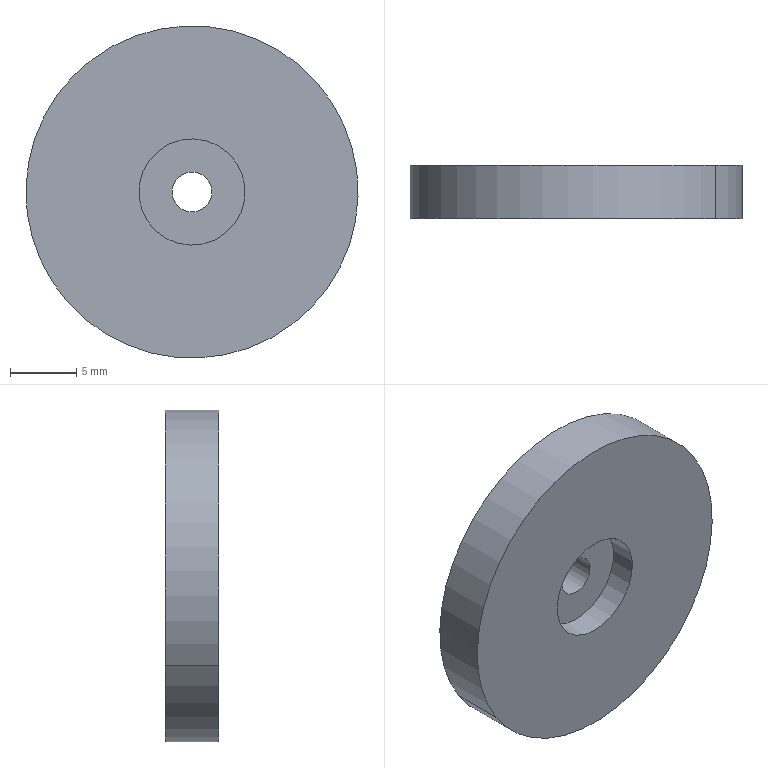Component | SolidWorks | EndCap4mm-3 | 1 solid | 9 faces | box 25 x 4 x 25 mm | volume 1849 mm3 | cylinder 6 | plane 3 | commonest cylinder face diameters 8 x2 25 x2 3 x2 | material 5454-O
build123d program:
from build123d import *

# Parameters (mm, degrees)
SKETCH1_R           = 12.5
SKETCH1_R_2         = 1.5
BOSS_EXTRUDE1_DEPTH = 4
SKETCH2_R           = 4
CUT_EXTRUDE1_DEPTH  = 2


with BuildPart() as part:
    # Sketch1 → Boss-Extrude1 (new body)
    with BuildSketch(Plane.XY):
        Circle(SKETCH1_R)
        Circle(SKETCH1_R_2, mode=Mode.SUBTRACT)
    extrude(amount=BOSS_EXTRUDE1_DEPTH)

    # Sketch2 → Cut-Extrude1 (cut)
    with BuildSketch(Plane.XY.offset(4)):
        Circle(SKETCH2_R)
    extrude(amount=-CUT_EXTRUDE1_DEPTH, mode=Mode.SUBTRACT)


solid = part.part

# Placed as in the assembly
solid = solid.moved(Location((6.846, 48.266, -166.507), (90, 0, 0)))
STEP:
#1=COLOUR_RGB('',0.7922,0.8196,0.9333);
#2=FILL_AREA_STYLE_COLOUR('',#1);
#3=FILL_AREA_STYLE('',(#2));
#4=SURFACE_STYLE_FILL_AREA(#3);
#5=SURFACE_SIDE_STYLE('',(#4));
#6=SURFACE_STYLE_USAGE(.BOTH.,#5);
#7=PRESENTATION_STYLE_ASSIGNMENT((#6));
#8=CARTESIAN_POINT('',(0.137,1.821,-6.641));
#9=VERTEX_POINT('',#8);
#10=CARTESIAN_POINT('',(0.402,1.821,-6.47));
#11=VERTEX_POINT('',#10);
#12=CARTESIAN_POINT('',(0.2695,1.821,-6.555));
#13=DIRECTION('',(-0.,-1.,-0.));
#14=DIRECTION('',(0.8414,0.,0.5405));
#15=AXIS2_PLACEMENT_3D('',#12,#13,#14);
#16=CIRCLE('',#15,0.1575);
#17=EDGE_CURVE('',#9,#11,#16,.T.);
#18=ORIENTED_EDGE('',*,*,#17,.F.);
#19=CARTESIAN_POINT('',(0.137,1.743,-6.641));
#20=VERTEX_POINT('',#19);
#21=CARTESIAN_POINT('',(0.137,1.821,-6.641));
#22=DIRECTION('',(-0.,-1.,-0.));
#23=VECTOR('',#22,39.37);
#24=LINE('',#21,#23);
#25=EDGE_CURVE('',#9,#20,#24,.T.);
#26=ORIENTED_EDGE('',*,*,#25,.T.);
#27=CARTESIAN_POINT('',(0.402,1.743,-6.47));
#28=VERTEX_POINT('',#27);
#29=CARTESIAN_POINT('',(0.2695,1.743,-6.555));
#30=DIRECTION('',(-0.,-1.,-0.));
#31=DIRECTION('',(0.8414,0.,0.5405));
#32=AXIS2_PLACEMENT_3D('',#29,#30,#31);
#33=CIRCLE('',#32,0.1575);
#34=EDGE_CURVE('',#20,#28,#33,.T.);
#35=ORIENTED_EDGE('',*,*,#34,.T.);
#36=CARTESIAN_POINT('',(0.402,1.821,-6.47));
#37=DIRECTION('',(-0.,-1.,-0.));
#38=VECTOR('',#37,39.37);
#39=LINE('',#36,#38);
#40=EDGE_CURVE('',#11,#28,#39,.T.);
#41=ORIENTED_EDGE('',*,*,#40,.F.);
#42=EDGE_LOOP('',(#18,#26,#35,#41));
#43=FACE_OUTER_BOUND('',#42,.T.);
#44=CARTESIAN_POINT('',(0.2695,1.821,-6.555));
#45=DIRECTION('',(-0.,-1.,-0.));
#46=DIRECTION('',(0.8414,0.,0.5405));
#47=AXIS2_PLACEMENT_3D('',#44,#45,#46);
#48=CYLINDRICAL_SURFACE('',#47,0.1575);
#49=ADVANCED_FACE('',(#43),#48,.F.);
#50=CARTESIAN_POINT('',(0.6836,1.743,-6.289));
#51=VERTEX_POINT('',#50);
#52=CARTESIAN_POINT('',(-0.1445,1.743,-6.821));
#53=VERTEX_POINT('',#52);
#54=CARTESIAN_POINT('',(0.2695,1.743,-6.555));
#55=DIRECTION('',(-0.,-1.,-0.));
#56=DIRECTION('',(0.8414,0.,0.5405));
#57=AXIS2_PLACEMENT_3D('',#54,#55,#56);
#58=CIRCLE('',#57,0.4921);
#59=EDGE_CURVE('',#51,#53,#58,.T.);
#60=ORIENTED_EDGE('',*,*,#59,.F.);
#61=CARTESIAN_POINT('',(0.6836,1.9,-6.289));
#62=VERTEX_POINT('',#61);
#63=CARTESIAN_POINT('',(0.6836,1.743,-6.289));
#64=DIRECTION('',(0.,1.,0.));
#65=VECTOR('',#64,39.37);
#66=LINE('',#63,#65);
#67=EDGE_CURVE('',#51,#62,#66,.T.);
#68=ORIENTED_EDGE('',*,*,#67,.T.);
#69=CARTESIAN_POINT('',(-0.1445,1.9,-6.821));
#70=VERTEX_POINT('',#69);
#71=CARTESIAN_POINT('',(0.2695,1.9,-6.555));
#72=DIRECTION('',(-0.,-1.,-0.));
#73=DIRECTION('',(0.8414,0.,0.5405));
#74=AXIS2_PLACEMENT_3D('',#71,#72,#73);
#75=CIRCLE('',#74,0.4921);
#76=EDGE_CURVE('',#62,#70,#75,.T.);
#77=ORIENTED_EDGE('',*,*,#76,.T.);
#78=CARTESIAN_POINT('',(-0.1445,1.743,-6.821));
#79=DIRECTION('',(0.,1.,0.));
#80=VECTOR('',#79,39.37);
#81=LINE('',#78,#80);
#82=EDGE_CURVE('',#53,#70,#81,.T.);
#83=ORIENTED_EDGE('',*,*,#82,.F.);
#84=EDGE_LOOP('',(#60,#68,#77,#83));
#85=FACE_OUTER_BOUND('',#84,.T.);
#86=CARTESIAN_POINT('',(0.2695,1.743,-6.555));
#87=DIRECTION('',(0.,1.,0.));
#88=DIRECTION('',(-0.8414,0.,-0.5405));
#89=AXIS2_PLACEMENT_3D('',#86,#87,#88);
#90=CYLINDRICAL_SURFACE('',#89,0.4921);
#91=ADVANCED_FACE('',(#85),#90,.T.);
#92=CARTESIAN_POINT('',(0.2198,1.821,-6.587));
#93=VERTEX_POINT('',#92);
#94=CARTESIAN_POINT('',(0.3192,1.821,-6.523));
#95=VERTEX_POINT('',#94);
#96=CARTESIAN_POINT('',(0.2695,1.821,-6.555));
#97=DIRECTION('',(-0.,-1.,-0.));
#98=DIRECTION('',(0.8414,0.,0.5405));
#99=AXIS2_PLACEMENT_3D('',#96,#97,#98);
#100=CIRCLE('',#99,0.05906);
#101=EDGE_CURVE('',#93,#95,#100,.T.);
#102=ORIENTED_EDGE('',*,*,#101,.T.);
#103=CARTESIAN_POINT('',(0.3192,1.9,-6.523));
#104=VERTEX_POINT('',#103);
#105=CARTESIAN_POINT('',(0.3192,1.743,-6.523));
#106=DIRECTION('',(0.,1.,0.));
#107=VECTOR('',#106,39.37);
#108=LINE('',#105,#107);
#109=EDGE_CURVE('',#95,#104,#108,.T.);
#110=ORIENTED_EDGE('',*,*,#109,.T.);
#111=CARTESIAN_POINT('',(0.2198,1.9,-6.587));
#112=VERTEX_POINT('',#111);
#113=CARTESIAN_POINT('',(0.2695,1.9,-6.555));
#114=DIRECTION('',(-0.,-1.,-0.));
#115=DIRECTION('',(0.8414,0.,0.5405));
#116=AXIS2_PLACEMENT_3D('',#113,#114,#115);
#117=CIRCLE('',#116,0.05906);
#118=EDGE_CURVE('',#112,#104,#117,.T.);
#119=ORIENTED_EDGE('',*,*,#118,.F.);
#120=CARTESIAN_POINT('',(0.2198,1.743,-6.587));
#121=DIRECTION('',(0.,1.,0.));
#122=VECTOR('',#121,39.37);
#123=LINE('',#120,#122);
#124=EDGE_CURVE('',#93,#112,#123,.T.);
#125=ORIENTED_EDGE('',*,*,#124,.F.);
#126=EDGE_LOOP('',(#102,#110,#119,#125));
#127=FACE_OUTER_BOUND('',#126,.T.);
#128=CARTESIAN_POINT('',(0.2695,1.743,-6.555));
#129=DIRECTION('',(0.,1.,0.));
#130=DIRECTION('',(-0.8414,0.,-0.5405));
#131=AXIS2_PLACEMENT_3D('',#128,#129,#130);
#132=CYLINDRICAL_SURFACE('',#131,0.05906);
#133=ADVANCED_FACE('',(#127),#132,.F.);
#134=ORIENTED_EDGE('',*,*,#109,.F.);
#135=CARTESIAN_POINT('',(0.2695,1.821,-6.555));
#136=DIRECTION('',(-0.,-1.,-0.));
#137=DIRECTION('',(0.8414,0.,0.5405));
#138=AXIS2_PLACEMENT_3D('',#135,#136,#137);
#139=CIRCLE('',#138,0.05906);
#140=EDGE_CURVE('',#95,#93,#139,.T.);
#141=ORIENTED_EDGE('',*,*,#140,.T.);
#142=ORIENTED_EDGE('',*,*,#124,.T.);
#143=CARTESIAN_POINT('',(0.2695,1.9,-6.555));
#144=DIRECTION('',(-0.,-1.,-0.));
#145=DIRECTION('',(0.8414,0.,0.5405));
#146=AXIS2_PLACEMENT_3D('',#143,#144,#145);
#147=CIRCLE('',#146,0.05906);
#148=EDGE_CURVE('',#104,#112,#147,.T.);
#149=ORIENTED_EDGE('',*,*,#148,.F.);
#150=EDGE_LOOP('',(#134,#141,#142,#149));
#151=FACE_OUTER_BOUND('',#150,.T.);
#152=CARTESIAN_POINT('',(0.2695,1.743,-6.555));
#153=DIRECTION('',(0.,1.,0.));
#154=DIRECTION('',(-0.8414,0.,-0.5405));
#155=AXIS2_PLACEMENT_3D('',#152,#153,#154);
#156=CYLINDRICAL_SURFACE('',#155,0.05906);
#157=ADVANCED_FACE('',(#151),#156,.F.);
#158=CARTESIAN_POINT('',(0.2695,1.743,-6.555));
#159=DIRECTION('',(-0.,-1.,-0.));
#160=DIRECTION('',(0.8414,0.,0.5405));
#161=AXIS2_PLACEMENT_3D('',#158,#159,#160);
#162=CIRCLE('',#161,0.1575);
#163=EDGE_CURVE('',#28,#20,#162,.T.);
#164=ORIENTED_EDGE('',*,*,#163,.F.);
#165=ORIENTED_EDGE('',*,*,#34,.F.);
#166=EDGE_LOOP('',(#164,#165));
#167=FACE_BOUND('',#166,.T.);
#168=CARTESIAN_POINT('',(0.2695,1.743,-6.555));
#169=DIRECTION('',(-0.,-1.,-0.));
#170=DIRECTION('',(0.8414,0.,0.5405));
#171=AXIS2_PLACEMENT_3D('',#168,#169,#170);
#172=CIRCLE('',#171,0.4921);
#173=EDGE_CURVE('',#53,#51,#172,.T.);
#174=ORIENTED_EDGE('',*,*,#173,.T.);
#175=ORIENTED_EDGE('',*,*,#59,.T.);
#176=EDGE_LOOP('',(#174,#175));
#177=FACE_OUTER_BOUND('',#176,.T.);
#178=CARTESIAN_POINT('',(0.2695,1.743,-6.555));
#179=DIRECTION('',(-0.,-1.,-0.));
#180=DIRECTION('',(0.8414,-0.,0.5405));
#181=AXIS2_PLACEMENT_3D('',#178,#179,#180);
#182=PLANE('',#181);
#183=ADVANCED_FACE('',(#167,#177),#182,.T.);
#184=CARTESIAN_POINT('',(0.2695,1.9,-6.555));
#185=DIRECTION('',(-0.,-1.,-0.));
#186=DIRECTION('',(0.8414,0.,0.5405));
#187=AXIS2_PLACEMENT_3D('',#184,#185,#186);
#188=CIRCLE('',#187,0.4921);
#189=EDGE_CURVE('',#70,#62,#188,.T.);
#190=ORIENTED_EDGE('',*,*,#189,.F.);
#191=ORIENTED_EDGE('',*,*,#76,.F.);
#192=EDGE_LOOP('',(#190,#191));
#193=FACE_OUTER_BOUND('',#192,.T.);
#194=ORIENTED_EDGE('',*,*,#118,.T.);
#195=ORIENTED_EDGE('',*,*,#148,.T.);
#196=EDGE_LOOP('',(#194,#195));
#197=FACE_BOUND('',#196,.T.);
#198=CARTESIAN_POINT('',(0.2695,1.9,-6.555));
#199=DIRECTION('',(-0.,-1.,-0.));
#200=DIRECTION('',(0.8414,-0.,0.5405));
#201=AXIS2_PLACEMENT_3D('',#198,#199,#200);
#202=PLANE('',#201);
#203=ADVANCED_FACE('',(#193,#197),#202,.F.);
#204=ORIENTED_EDGE('',*,*,#67,.F.);
#205=ORIENTED_EDGE('',*,*,#173,.F.);
#206=ORIENTED_EDGE('',*,*,#82,.T.);
#207=ORIENTED_EDGE('',*,*,#189,.T.);
#208=EDGE_LOOP('',(#204,#205,#206,#207));
#209=FACE_OUTER_BOUND('',#208,.T.);
#210=CARTESIAN_POINT('',(0.2695,1.743,-6.555));
#211=DIRECTION('',(0.,1.,0.));
#212=DIRECTION('',(-0.8414,0.,-0.5405));
#213=AXIS2_PLACEMENT_3D('',#210,#211,#212);
#214=CYLINDRICAL_SURFACE('',#213,0.4921);
#215=ADVANCED_FACE('',(#209),#214,.T.);
#216=ORIENTED_EDGE('',*,*,#25,.F.);
#217=CARTESIAN_POINT('',(0.2695,1.821,-6.555));
#218=DIRECTION('',(-0.,-1.,-0.));
#219=DIRECTION('',(0.8414,0.,0.5405));
#220=AXIS2_PLACEMENT_3D('',#217,#218,#219);
#221=CIRCLE('',#220,0.1575);
#222=EDGE_CURVE('',#11,#9,#221,.T.);
#223=ORIENTED_EDGE('',*,*,#222,.F.);
#224=ORIENTED_EDGE('',*,*,#40,.T.);
#225=ORIENTED_EDGE('',*,*,#163,.T.);
#226=EDGE_LOOP('',(#216,#223,#224,#225));
#227=FACE_OUTER_BOUND('',#226,.T.);
#228=CARTESIAN_POINT('',(0.2695,1.821,-6.555));
#229=DIRECTION('',(-0.,-1.,-0.));
#230=DIRECTION('',(0.8414,0.,0.5405));
#231=AXIS2_PLACEMENT_3D('',#228,#229,#230);
#232=CYLINDRICAL_SURFACE('',#231,0.1575);
#233=ADVANCED_FACE('',(#227),#232,.F.);
#234=ORIENTED_EDGE('',*,*,#101,.F.);
#235=ORIENTED_EDGE('',*,*,#140,.F.);
#236=EDGE_LOOP('',(#234,#235));
#237=FACE_BOUND('',#236,.T.);
#238=ORIENTED_EDGE('',*,*,#222,.T.);
#239=ORIENTED_EDGE('',*,*,#17,.T.);
#240=EDGE_LOOP('',(#238,#239));
#241=FACE_OUTER_BOUND('',#240,.T.);
#242=CARTESIAN_POINT('',(0.2695,1.821,-6.555));
#243=DIRECTION('',(-0.,-1.,-0.));
#244=DIRECTION('',(0.8414,-0.,0.5405));
#245=AXIS2_PLACEMENT_3D('',#242,#243,#244);
#246=PLANE('',#245);
#247=ADVANCED_FACE('',(#237,#241),#246,.T.);
#248=CLOSED_SHELL('',(#49,#91,#133,#157,#183,#203,#215,#233,#247));
#249=MANIFOLD_SOLID_BREP('',#248);
#250=STYLED_ITEM('',(#7),#249);
#251=(LENGTH_UNIT()NAMED_UNIT(*)SI_UNIT($,.METRE.));
#252=LENGTH_MEASURE_WITH_UNIT(LENGTH_MEASURE(0.0254),#251);
#253=DIMENSIONAL_EXPONENTS(1.,0.,0.,0.,0.,0.,0.);
#254=(CONVERSION_BASED_UNIT('',#252)LENGTH_UNIT()NAMED_UNIT(#253));
#255=UNCERTAINTY_MEASURE_WITH_UNIT(LENGTH_MEASURE(0.00001),#254,'','');
#256=(NAMED_UNIT(*)PLANE_ANGLE_UNIT()SI_UNIT($,.RADIAN.));
#257=(NAMED_UNIT(*)SI_UNIT($,.STERADIAN.)SOLID_ANGLE_UNIT());
#258=(GEOMETRIC_REPRESENTATION_CONTEXT(3)GLOBAL_UNCERTAINTY_ASSIGNED_CONTEXT((#255))GLOBAL_UNIT_ASSIGNED_CONTEXT((#254,#256,#257))REPRESENTATION_CONTEXT('',''));
#259=MECHANICAL_DESIGN_GEOMETRIC_PRESENTATION_REPRESENTATION('',(#250),#258);
#260=PRESENTATION_LAYER_ASSIGNMENT('','',(#250));
#261=CARTESIAN_POINT('',(0.,0.,0.));
#262=DIRECTION('',(0.,0.,1.));
#263=DIRECTION('',(1.,0.,0.));
#264=AXIS2_PLACEMENT_3D('',#261,#262,#263);
#265=(LENGTH_UNIT()NAMED_UNIT(*)SI_UNIT($,.METRE.));
#266=LENGTH_MEASURE_WITH_UNIT(LENGTH_MEASURE(0.0254),#265);
#267=DIMENSIONAL_EXPONENTS(1.,0.,0.,0.,0.,0.,0.);
#268=(CONVERSION_BASED_UNIT('',#266)LENGTH_UNIT()NAMED_UNIT(#267));
#269=UNCERTAINTY_MEASURE_WITH_UNIT(LENGTH_MEASURE(0.00001),#268,'','');
#270=(NAMED_UNIT(*)PLANE_ANGLE_UNIT()SI_UNIT($,.RADIAN.));
#271=(NAMED_UNIT(*)SI_UNIT($,.STERADIAN.)SOLID_ANGLE_UNIT());
#272=(GEOMETRIC_REPRESENTATION_CONTEXT(3)GLOBAL_UNCERTAINTY_ASSIGNED_CONTEXT((#269))GLOBAL_UNIT_ASSIGNED_CONTEXT((#268,#270,#271))REPRESENTATION_CONTEXT('',''));
#273=ADVANCED_BREP_SHAPE_REPRESENTATION('',(#249,#264),#272);